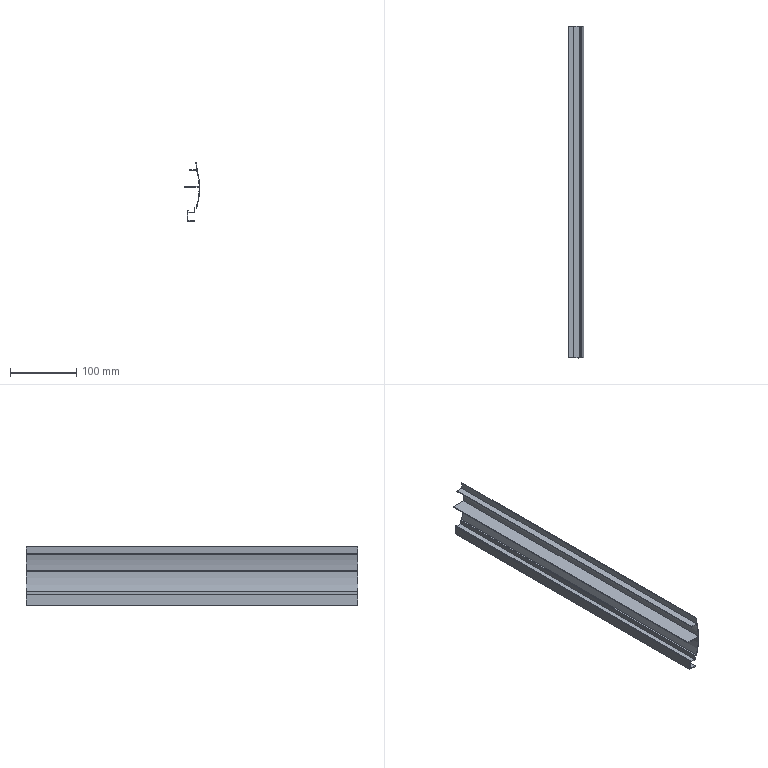Component | SolidWorks | Blade-17 | 1 solid | 27 faces | box 23.47 x 500 x 87.98 mm | volume 81818 mm3 | plane 24 | cylinder 3 | commonest cylinder face diameters 190.922 x3
build123d program:
from build123d import *

# Parameters (mm, degrees)
BOSS_EXTRUDE1_DEPTH = 500


with BuildPart() as part:
    # Sketch1 → Boss-Extrude1 (new body)
    with BuildSketch(Plane.XY):
        with BuildLine():
            Line((52.448, 10.612), (52.448, -5.008))
            Line((52.448, -5.008), (51.164, -5.008))
            Line((51.164, -5.008), (51.164, 10.227))
            Line((51.164, 10.227), (51.164, 17.359))
            ThreePointArc((51.164, 17.359), (35.594, 16.542), (20.364, 13.201))
            Line((20.364, 13.201), (20.364, 10.4))
            Line((20.364, 10.4), (13.6, 10.4))
            Line((13.6, 10.4), (13.6, 1.1))
            Line((13.6, 1.1), (15.3, 1.1))
            Line((15.3, 1.1), (15.3, 0))
            Line((15.3, 0), (0, 0))
            Line((0, 0), (0, 11.2))
            Line((0, 11.2), (1.1, 11.2))
            Line((1.1, 11.2), (1.1, 1.1))
            Line((1.1, 1.1), (12.5, 1.1))
            Line((12.5, 1.1), (12.5, 11.5))
            Line((12.5, 11.5), (19.4, 11.5))
            Line((19.4, 11.5), (19.4, 14))
            ThreePointArc((19.4, 14), (48.454, 18.5), (77.5, 13.945))
            Line((77.5, 13.945), (88, 12.9))
            Line((88, 12.9), (88, 11.8))
            Line((88, 11.8), (77.5, 12.9))
            Line((77.5, 12.9), (77.5, 2.6))
            Line((77.5, 2.6), (76.4, 2.6))
            Line((76.4, 2.6), (76.4, 13.19))
            ThreePointArc((76.4, 13.19), (64.556, 16.017), (52.448, 17.313))
            Line((52.448, 17.313), (52.448, 10.612))
        make_face()
    extrude(amount=BOSS_EXTRUDE1_DEPTH)


solid = part.part

# Placed as in the assembly
solid = solid.moved(Location((101.142, 41.806, 695.913), (-90, 0, -89.089)))
STEP:
#1=COLOUR_RGB('',0.7922,0.8196,0.9333);
#2=FILL_AREA_STYLE_COLOUR('',#1);
#3=FILL_AREA_STYLE('',(#2));
#4=SURFACE_STYLE_FILL_AREA(#3);
#5=SURFACE_SIDE_STYLE('',(#4));
#6=SURFACE_STYLE_USAGE(.BOTH.,#5);
#7=PRESENTATION_STYLE_ASSIGNMENT((#6));
#8=CARTESIAN_POINT('',(4.549,1.646,30.397));
#9=VERTEX_POINT('',#8);
#10=CARTESIAN_POINT('',(4.696,1.646,29.452));
#11=VERTEX_POINT('',#10);
#12=CARTESIAN_POINT('',(0.9394,1.646,29.351));
#13=DIRECTION('',(-0.,1.,0.));
#14=DIRECTION('',(0.0159,-0.,0.9999));
#15=AXIS2_PLACEMENT_3D('',#12,#13,#14);
#16=CIRCLE('',#15,3.758);
#17=EDGE_CURVE('',#9,#11,#16,.T.);
#18=ORIENTED_EDGE('',*,*,#17,.F.);
#19=CARTESIAN_POINT('',(4.549,21.331,30.397));
#20=VERTEX_POINT('',#19);
#21=CARTESIAN_POINT('',(4.549,21.331,30.397));
#22=DIRECTION('',(0.,-1.,-0.));
#23=VECTOR('',#22,39.37);
#24=LINE('',#21,#23);
#25=EDGE_CURVE('',#20,#9,#24,.T.);
#26=ORIENTED_EDGE('',*,*,#25,.F.);
#27=CARTESIAN_POINT('',(4.696,21.331,29.452));
#28=VERTEX_POINT('',#27);
#29=CARTESIAN_POINT('',(0.9394,21.331,29.351));
#30=DIRECTION('',(-0.,1.,0.));
#31=DIRECTION('',(0.0159,0.,0.9999));
#32=AXIS2_PLACEMENT_3D('',#29,#30,#31);
#33=CIRCLE('',#32,3.758);
#34=EDGE_CURVE('',#20,#28,#33,.T.);
#35=ORIENTED_EDGE('',*,*,#34,.T.);
#36=CARTESIAN_POINT('',(4.696,21.331,29.452));
#37=DIRECTION('',(0.,-1.,-0.));
#38=VECTOR('',#37,39.37);
#39=LINE('',#36,#38);
#40=EDGE_CURVE('',#28,#11,#39,.T.);
#41=ORIENTED_EDGE('',*,*,#40,.T.);
#42=EDGE_LOOP('',(#18,#26,#35,#41));
#43=FACE_OUTER_BOUND('',#42,.T.);
#44=CARTESIAN_POINT('',(0.9394,21.331,29.351));
#45=DIRECTION('',(0.,-1.,-0.));
#46=DIRECTION('',(-0.0159,0.,-0.9999));
#47=AXIS2_PLACEMENT_3D('',#44,#45,#46);
#48=CYLINDRICAL_SURFACE('',#47,3.758);
#49=ADVANCED_FACE('',(#43),#48,.F.);
#50=CARTESIAN_POINT('',(4.132,1.646,30.404));
#51=VERTEX_POINT('',#50);
#52=CARTESIAN_POINT('',(4.549,1.646,30.397));
#53=DIRECTION('',(-0.9999,-0.,0.0159));
#54=VECTOR('',#53,39.37);
#55=LINE('',#52,#54);
#56=EDGE_CURVE('',#9,#51,#55,.T.);
#57=ORIENTED_EDGE('',*,*,#56,.T.);
#58=CARTESIAN_POINT('',(4.132,21.331,30.404));
#59=VERTEX_POINT('',#58);
#60=CARTESIAN_POINT('',(4.132,21.331,30.404));
#61=DIRECTION('',(0.,-1.,-0.));
#62=VECTOR('',#61,39.37);
#63=LINE('',#60,#62);
#64=EDGE_CURVE('',#59,#51,#63,.T.);
#65=ORIENTED_EDGE('',*,*,#64,.F.);
#66=CARTESIAN_POINT('',(4.549,21.331,30.397));
#67=DIRECTION('',(-0.9999,-0.,0.0159));
#68=VECTOR('',#67,39.37);
#69=LINE('',#66,#68);
#70=EDGE_CURVE('',#20,#59,#69,.T.);
#71=ORIENTED_EDGE('',*,*,#70,.F.);
#72=ORIENTED_EDGE('',*,*,#25,.T.);
#73=EDGE_LOOP('',(#57,#65,#71,#72));
#74=FACE_OUTER_BOUND('',#73,.T.);
#75=CARTESIAN_POINT('',(4.549,21.331,30.397));
#76=DIRECTION('',(0.0159,-0.,0.9999));
#77=DIRECTION('',(0.,-1.,-0.));
#78=AXIS2_PLACEMENT_3D('',#75,#76,#77);
#79=PLANE('',#78);
#80=ADVANCED_FACE('',(#74),#79,.F.);
#81=CARTESIAN_POINT('',(4.133,1.646,30.447));
#82=VERTEX_POINT('',#81);
#83=CARTESIAN_POINT('',(4.132,1.646,30.404));
#84=DIRECTION('',(0.0159,-0.,0.9999));
#85=VECTOR('',#84,39.37);
#86=LINE('',#83,#85);
#87=EDGE_CURVE('',#51,#82,#86,.T.);
#88=ORIENTED_EDGE('',*,*,#87,.T.);
#89=CARTESIAN_POINT('',(4.133,21.331,30.447));
#90=VERTEX_POINT('',#89);
#91=CARTESIAN_POINT('',(4.133,21.331,30.447));
#92=DIRECTION('',(0.,-1.,-0.));
#93=VECTOR('',#92,39.37);
#94=LINE('',#91,#93);
#95=EDGE_CURVE('',#90,#82,#94,.T.);
#96=ORIENTED_EDGE('',*,*,#95,.F.);
#97=CARTESIAN_POINT('',(4.132,21.331,30.404));
#98=DIRECTION('',(0.0159,-0.,0.9999));
#99=VECTOR('',#98,39.37);
#100=LINE('',#97,#99);
#101=EDGE_CURVE('',#59,#90,#100,.T.);
#102=ORIENTED_EDGE('',*,*,#101,.F.);
#103=ORIENTED_EDGE('',*,*,#64,.T.);
#104=EDGE_LOOP('',(#88,#96,#102,#103));
#105=FACE_OUTER_BOUND('',#104,.T.);
#106=CARTESIAN_POINT('',(4.132,21.331,30.404));
#107=DIRECTION('',(0.9999,0.,-0.0159));
#108=DIRECTION('',(-0.,1.,0.));
#109=AXIS2_PLACEMENT_3D('',#106,#107,#108);
#110=PLANE('',#109);
#111=ADVANCED_FACE('',(#105),#110,.F.);
#112=CARTESIAN_POINT('',(4.538,1.646,30.441));
#113=VERTEX_POINT('',#112);
#114=CARTESIAN_POINT('',(4.133,1.646,30.447));
#115=DIRECTION('',(0.9999,0.,-0.0159));
#116=VECTOR('',#115,39.37);
#117=LINE('',#114,#116);
#118=EDGE_CURVE('',#82,#113,#117,.T.);
#119=ORIENTED_EDGE('',*,*,#118,.T.);
#120=CARTESIAN_POINT('',(4.538,21.331,30.441));
#121=VERTEX_POINT('',#120);
#122=CARTESIAN_POINT('',(4.538,21.331,30.441));
#123=DIRECTION('',(0.,-1.,-0.));
#124=VECTOR('',#123,39.37);
#125=LINE('',#122,#124);
#126=EDGE_CURVE('',#121,#113,#125,.T.);
#127=ORIENTED_EDGE('',*,*,#126,.F.);
#128=CARTESIAN_POINT('',(4.133,21.331,30.447));
#129=DIRECTION('',(0.9999,0.,-0.0159));
#130=VECTOR('',#129,39.37);
#131=LINE('',#128,#130);
#132=EDGE_CURVE('',#90,#121,#131,.T.);
#133=ORIENTED_EDGE('',*,*,#132,.F.);
#134=ORIENTED_EDGE('',*,*,#95,.T.);
#135=EDGE_LOOP('',(#119,#127,#133,#134));
#136=FACE_OUTER_BOUND('',#135,.T.);
#137=CARTESIAN_POINT('',(4.133,21.331,30.447));
#138=DIRECTION('',(-0.0159,0.,-0.9999));
#139=DIRECTION('',(-0.,1.,0.));
#140=AXIS2_PLACEMENT_3D('',#137,#138,#139);
#141=PLANE('',#140);
#142=ADVANCED_FACE('',(#136),#141,.F.);
#143=CARTESIAN_POINT('',(4.502,1.646,30.855));
#144=VERTEX_POINT('',#143);
#145=CARTESIAN_POINT('',(4.538,1.646,30.441));
#146=DIRECTION('',(-0.08837,-0.,0.9961));
#147=VECTOR('',#146,39.37);
#148=LINE('',#145,#147);
#149=EDGE_CURVE('',#113,#144,#148,.T.);
#150=ORIENTED_EDGE('',*,*,#149,.T.);
#151=CARTESIAN_POINT('',(4.502,21.331,30.855));
#152=VERTEX_POINT('',#151);
#153=CARTESIAN_POINT('',(4.502,21.331,30.855));
#154=DIRECTION('',(0.,-1.,-0.));
#155=VECTOR('',#154,39.37);
#156=LINE('',#153,#155);
#157=EDGE_CURVE('',#152,#144,#156,.T.);
#158=ORIENTED_EDGE('',*,*,#157,.F.);
#159=CARTESIAN_POINT('',(4.538,21.331,30.441));
#160=DIRECTION('',(-0.08837,-0.,0.9961));
#161=VECTOR('',#160,39.37);
#162=LINE('',#159,#161);
#163=EDGE_CURVE('',#121,#152,#162,.T.);
#164=ORIENTED_EDGE('',*,*,#163,.F.);
#165=ORIENTED_EDGE('',*,*,#126,.T.);
#166=EDGE_LOOP('',(#150,#158,#164,#165));
#167=FACE_OUTER_BOUND('',#166,.T.);
#168=CARTESIAN_POINT('',(4.538,21.331,30.441));
#169=DIRECTION('',(0.9961,0.,0.08837));
#170=DIRECTION('',(0.08837,0.,-0.9961));
#171=AXIS2_PLACEMENT_3D('',#168,#169,#170);
#172=PLANE('',#171);
#173=ADVANCED_FACE('',(#167),#172,.F.);
#174=CARTESIAN_POINT('',(4.545,1.646,30.854));
#175=VERTEX_POINT('',#174);
#176=CARTESIAN_POINT('',(4.502,1.646,30.855));
#177=DIRECTION('',(0.9999,0.,-0.0159));
#178=VECTOR('',#177,39.37);
#179=LINE('',#176,#178);
#180=EDGE_CURVE('',#144,#175,#179,.T.);
#181=ORIENTED_EDGE('',*,*,#180,.T.);
#182=CARTESIAN_POINT('',(4.545,21.331,30.854));
#183=VERTEX_POINT('',#182);
#184=CARTESIAN_POINT('',(4.545,21.331,30.854));
#185=DIRECTION('',(0.,-1.,-0.));
#186=VECTOR('',#185,39.37);
#187=LINE('',#184,#186);
#188=EDGE_CURVE('',#183,#175,#187,.T.);
#189=ORIENTED_EDGE('',*,*,#188,.F.);
#190=CARTESIAN_POINT('',(4.502,21.331,30.855));
#191=DIRECTION('',(0.9999,0.,-0.0159));
#192=VECTOR('',#191,39.37);
#193=LINE('',#190,#192);
#194=EDGE_CURVE('',#152,#183,#193,.T.);
#195=ORIENTED_EDGE('',*,*,#194,.F.);
#196=ORIENTED_EDGE('',*,*,#157,.T.);
#197=EDGE_LOOP('',(#181,#189,#195,#196));
#198=FACE_OUTER_BOUND('',#197,.T.);
#199=CARTESIAN_POINT('',(4.502,21.331,30.855));
#200=DIRECTION('',(-0.0159,0.,-0.9999));
#201=DIRECTION('',(-0.,1.,0.));
#202=AXIS2_PLACEMENT_3D('',#199,#200,#201);
#203=PLANE('',#202);
#204=ADVANCED_FACE('',(#198),#203,.F.);
#205=CARTESIAN_POINT('',(4.579,1.646,30.44));
#206=VERTEX_POINT('',#205);
#207=CARTESIAN_POINT('',(4.545,1.646,30.854));
#208=DIRECTION('',(0.08323,0.,-0.9965));
#209=VECTOR('',#208,39.37);
#210=LINE('',#207,#209);
#211=EDGE_CURVE('',#175,#206,#210,.T.);
#212=ORIENTED_EDGE('',*,*,#211,.T.);
#213=CARTESIAN_POINT('',(4.579,21.331,30.44));
#214=VERTEX_POINT('',#213);
#215=CARTESIAN_POINT('',(4.579,21.331,30.44));
#216=DIRECTION('',(0.,-1.,-0.));
#217=VECTOR('',#216,39.37);
#218=LINE('',#215,#217);
#219=EDGE_CURVE('',#214,#206,#218,.T.);
#220=ORIENTED_EDGE('',*,*,#219,.F.);
#221=CARTESIAN_POINT('',(4.545,21.331,30.854));
#222=DIRECTION('',(0.08323,0.,-0.9965));
#223=VECTOR('',#222,39.37);
#224=LINE('',#221,#223);
#225=EDGE_CURVE('',#183,#214,#224,.T.);
#226=ORIENTED_EDGE('',*,*,#225,.F.);
#227=ORIENTED_EDGE('',*,*,#188,.T.);
#228=EDGE_LOOP('',(#212,#220,#226,#227));
#229=FACE_OUTER_BOUND('',#228,.T.);
#230=CARTESIAN_POINT('',(4.545,21.331,30.854));
#231=DIRECTION('',(-0.9965,-0.,-0.08323));
#232=DIRECTION('',(-0.08323,-0.,0.9965));
#233=AXIS2_PLACEMENT_3D('',#230,#231,#232);
#234=PLANE('',#233);
#235=ADVANCED_FACE('',(#229),#234,.F.);
#236=CARTESIAN_POINT('',(4.545,1.646,28.153));
#237=VERTEX_POINT('',#236);
#238=CARTESIAN_POINT('',(0.9827,1.646,29.35));
#239=DIRECTION('',(-0.,1.,0.));
#240=DIRECTION('',(0.0159,-0.,0.9999));
#241=AXIS2_PLACEMENT_3D('',#238,#239,#240);
#242=CIRCLE('',#241,3.758);
#243=EDGE_CURVE('',#206,#237,#242,.T.);
#244=ORIENTED_EDGE('',*,*,#243,.T.);
#245=CARTESIAN_POINT('',(4.545,21.331,28.153));
#246=VERTEX_POINT('',#245);
#247=CARTESIAN_POINT('',(4.545,21.331,28.153));
#248=DIRECTION('',(0.,-1.,-0.));
#249=VECTOR('',#248,39.37);
#250=LINE('',#247,#249);
#251=EDGE_CURVE('',#246,#237,#250,.T.);
#252=ORIENTED_EDGE('',*,*,#251,.F.);
#253=CARTESIAN_POINT('',(0.9827,21.331,29.35));
#254=DIRECTION('',(-0.,1.,0.));
#255=DIRECTION('',(0.0159,0.,0.9999));
#256=AXIS2_PLACEMENT_3D('',#253,#254,#255);
#257=CIRCLE('',#256,3.758);
#258=EDGE_CURVE('',#214,#246,#257,.T.);
#259=ORIENTED_EDGE('',*,*,#258,.F.);
#260=ORIENTED_EDGE('',*,*,#219,.T.);
#261=EDGE_LOOP('',(#244,#252,#259,#260));
#262=FACE_OUTER_BOUND('',#261,.T.);
#263=CARTESIAN_POINT('',(0.9827,21.331,29.35));
#264=DIRECTION('',(0.,-1.,-0.));
#265=DIRECTION('',(-0.0159,0.,-0.9999));
#266=AXIS2_PLACEMENT_3D('',#263,#264,#265);
#267=CYLINDRICAL_SURFACE('',#266,3.758);
#268=ADVANCED_FACE('',(#262),#267,.T.);
#269=CARTESIAN_POINT('',(4.447,1.646,28.155));
#270=VERTEX_POINT('',#269);
#271=CARTESIAN_POINT('',(4.545,1.646,28.153));
#272=DIRECTION('',(-0.9999,-0.,0.0159));
#273=VECTOR('',#272,39.37);
#274=LINE('',#271,#273);
#275=EDGE_CURVE('',#237,#270,#274,.T.);
#276=ORIENTED_EDGE('',*,*,#275,.T.);
#277=CARTESIAN_POINT('',(4.447,21.331,28.155));
#278=VERTEX_POINT('',#277);
#279=CARTESIAN_POINT('',(4.447,21.331,28.155));
#280=DIRECTION('',(0.,-1.,-0.));
#281=VECTOR('',#280,39.37);
#282=LINE('',#279,#281);
#283=EDGE_CURVE('',#278,#270,#282,.T.);
#284=ORIENTED_EDGE('',*,*,#283,.F.);
#285=CARTESIAN_POINT('',(4.545,21.331,28.153));
#286=DIRECTION('',(-0.9999,-0.,0.0159));
#287=VECTOR('',#286,39.37);
#288=LINE('',#285,#287);
#289=EDGE_CURVE('',#246,#278,#288,.T.);
#290=ORIENTED_EDGE('',*,*,#289,.F.);
#291=ORIENTED_EDGE('',*,*,#251,.T.);
#292=EDGE_LOOP('',(#276,#284,#290,#291));
#293=FACE_OUTER_BOUND('',#292,.T.);
#294=CARTESIAN_POINT('',(4.545,21.331,28.153));
#295=DIRECTION('',(0.0159,-0.,0.9999));
#296=DIRECTION('',(0.,-1.,-0.));
#297=AXIS2_PLACEMENT_3D('',#294,#295,#296);
#298=PLANE('',#297);
#299=ADVANCED_FACE('',(#293),#298,.F.);
#300=CARTESIAN_POINT('',(4.442,1.646,27.883));
#301=VERTEX_POINT('',#300);
#302=CARTESIAN_POINT('',(4.447,1.646,28.155));
#303=DIRECTION('',(-0.0159,0.,-0.9999));
#304=VECTOR('',#303,39.37);
#305=LINE('',#302,#304);
#306=EDGE_CURVE('',#270,#301,#305,.T.);
#307=ORIENTED_EDGE('',*,*,#306,.T.);
#308=CARTESIAN_POINT('',(4.442,21.331,27.883));
#309=VERTEX_POINT('',#308);
#310=CARTESIAN_POINT('',(4.442,21.331,27.883));
#311=DIRECTION('',(0.,-1.,-0.));
#312=VECTOR('',#311,39.37);
#313=LINE('',#310,#312);
#314=EDGE_CURVE('',#309,#301,#313,.T.);
#315=ORIENTED_EDGE('',*,*,#314,.F.);
#316=CARTESIAN_POINT('',(4.447,21.331,28.155));
#317=DIRECTION('',(-0.0159,0.,-0.9999));
#318=VECTOR('',#317,39.37);
#319=LINE('',#316,#318);
#320=EDGE_CURVE('',#278,#309,#319,.T.);
#321=ORIENTED_EDGE('',*,*,#320,.F.);
#322=ORIENTED_EDGE('',*,*,#283,.T.);
#323=EDGE_LOOP('',(#307,#315,#321,#322));
#324=FACE_OUTER_BOUND('',#323,.T.);
#325=CARTESIAN_POINT('',(4.447,21.331,28.155));
#326=DIRECTION('',(-0.9999,-0.,0.0159));
#327=DIRECTION('',(0.,-1.,-0.));
#328=AXIS2_PLACEMENT_3D('',#325,#326,#327);
#329=PLANE('',#328);
#330=ADVANCED_FACE('',(#324),#329,.F.);
#331=CARTESIAN_POINT('',(4.033,1.646,27.89));
#332=VERTEX_POINT('',#331);
#333=CARTESIAN_POINT('',(4.442,1.646,27.883));
#334=DIRECTION('',(-0.9999,-0.,0.0159));
#335=VECTOR('',#334,39.37);
#336=LINE('',#333,#335);
#337=EDGE_CURVE('',#301,#332,#336,.T.);
#338=ORIENTED_EDGE('',*,*,#337,.T.);
#339=CARTESIAN_POINT('',(4.033,21.331,27.89));
#340=VERTEX_POINT('',#339);
#341=CARTESIAN_POINT('',(4.033,21.331,27.89));
#342=DIRECTION('',(0.,-1.,-0.));
#343=VECTOR('',#342,39.37);
#344=LINE('',#341,#343);
#345=EDGE_CURVE('',#340,#332,#344,.T.);
#346=ORIENTED_EDGE('',*,*,#345,.F.);
#347=CARTESIAN_POINT('',(4.442,21.331,27.883));
#348=DIRECTION('',(-0.9999,-0.,0.0159));
#349=VECTOR('',#348,39.37);
#350=LINE('',#347,#349);
#351=EDGE_CURVE('',#309,#340,#350,.T.);
#352=ORIENTED_EDGE('',*,*,#351,.F.);
#353=ORIENTED_EDGE('',*,*,#314,.T.);
#354=EDGE_LOOP('',(#338,#346,#352,#353));
#355=FACE_OUTER_BOUND('',#354,.T.);
#356=CARTESIAN_POINT('',(4.442,21.331,27.883));
#357=DIRECTION('',(0.0159,-0.,0.9999));
#358=DIRECTION('',(0.,-1.,-0.));
#359=AXIS2_PLACEMENT_3D('',#356,#357,#358);
#360=PLANE('',#359);
#361=ADVANCED_FACE('',(#355),#360,.F.);
#362=CARTESIAN_POINT('',(4.026,1.646,27.441));
#363=VERTEX_POINT('',#362);
#364=CARTESIAN_POINT('',(4.033,1.646,27.89));
#365=DIRECTION('',(-0.0159,0.,-0.9999));
#366=VECTOR('',#365,39.37);
#367=LINE('',#364,#366);
#368=EDGE_CURVE('',#332,#363,#367,.T.);
#369=ORIENTED_EDGE('',*,*,#368,.T.);
#370=CARTESIAN_POINT('',(4.026,21.331,27.441));
#371=VERTEX_POINT('',#370);
#372=CARTESIAN_POINT('',(4.026,21.331,27.441));
#373=DIRECTION('',(0.,-1.,-0.));
#374=VECTOR('',#373,39.37);
#375=LINE('',#372,#374);
#376=EDGE_CURVE('',#371,#363,#375,.T.);
#377=ORIENTED_EDGE('',*,*,#376,.F.);
#378=CARTESIAN_POINT('',(4.033,21.331,27.89));
#379=DIRECTION('',(-0.0159,0.,-0.9999));
#380=VECTOR('',#379,39.37);
#381=LINE('',#378,#380);
#382=EDGE_CURVE('',#340,#371,#381,.T.);
#383=ORIENTED_EDGE('',*,*,#382,.F.);
#384=ORIENTED_EDGE('',*,*,#345,.T.);
#385=EDGE_LOOP('',(#369,#377,#383,#384));
#386=FACE_OUTER_BOUND('',#385,.T.);
#387=CARTESIAN_POINT('',(4.033,21.331,27.89));
#388=DIRECTION('',(-0.9999,-0.,0.0159));
#389=DIRECTION('',(0.,-1.,-0.));
#390=AXIS2_PLACEMENT_3D('',#387,#388,#389);
#391=PLANE('',#390);
#392=ADVANCED_FACE('',(#386),#391,.F.);
#393=CARTESIAN_POINT('',(4.424,1.646,27.434));
#394=VERTEX_POINT('',#393);
#395=CARTESIAN_POINT('',(4.026,1.646,27.441));
#396=DIRECTION('',(0.9999,0.,-0.0159));
#397=VECTOR('',#396,39.37);
#398=LINE('',#395,#397);
#399=EDGE_CURVE('',#363,#394,#398,.T.);
#400=ORIENTED_EDGE('',*,*,#399,.T.);
#401=CARTESIAN_POINT('',(4.424,21.331,27.434));
#402=VERTEX_POINT('',#401);
#403=CARTESIAN_POINT('',(4.424,21.331,27.434));
#404=DIRECTION('',(0.,-1.,-0.));
#405=VECTOR('',#404,39.37);
#406=LINE('',#403,#405);
#407=EDGE_CURVE('',#402,#394,#406,.T.);
#408=ORIENTED_EDGE('',*,*,#407,.F.);
#409=CARTESIAN_POINT('',(4.026,21.331,27.441));
#410=DIRECTION('',(0.9999,0.,-0.0159));
#411=VECTOR('',#410,39.37);
#412=LINE('',#409,#411);
#413=EDGE_CURVE('',#371,#402,#412,.T.);
#414=ORIENTED_EDGE('',*,*,#413,.F.);
#415=ORIENTED_EDGE('',*,*,#376,.T.);
#416=EDGE_LOOP('',(#400,#408,#414,#415));
#417=FACE_OUTER_BOUND('',#416,.T.);
#418=CARTESIAN_POINT('',(4.026,21.331,27.441));
#419=DIRECTION('',(-0.0159,0.,-0.9999));
#420=DIRECTION('',(-0.,1.,0.));
#421=AXIS2_PLACEMENT_3D('',#418,#419,#420);
#422=PLANE('',#421);
#423=ADVANCED_FACE('',(#417),#422,.F.);
#424=CARTESIAN_POINT('',(4.423,1.646,27.391));
#425=VERTEX_POINT('',#424);
#426=CARTESIAN_POINT('',(4.424,1.646,27.434));
#427=DIRECTION('',(-0.0159,0.,-0.9999));
#428=VECTOR('',#427,39.37);
#429=LINE('',#426,#428);
#430=EDGE_CURVE('',#394,#425,#429,.T.);
#431=ORIENTED_EDGE('',*,*,#430,.T.);
#432=CARTESIAN_POINT('',(4.423,21.331,27.391));
#433=VERTEX_POINT('',#432);
#434=CARTESIAN_POINT('',(4.423,21.331,27.391));
#435=DIRECTION('',(0.,-1.,-0.));
#436=VECTOR('',#435,39.37);
#437=LINE('',#434,#436);
#438=EDGE_CURVE('',#433,#425,#437,.T.);
#439=ORIENTED_EDGE('',*,*,#438,.F.);
#440=CARTESIAN_POINT('',(4.424,21.331,27.434));
#441=DIRECTION('',(-0.0159,0.,-0.9999));
#442=VECTOR('',#441,39.37);
#443=LINE('',#440,#442);
#444=EDGE_CURVE('',#402,#433,#443,.T.);
#445=ORIENTED_EDGE('',*,*,#444,.F.);
#446=ORIENTED_EDGE('',*,*,#407,.T.);
#447=EDGE_LOOP('',(#431,#439,#445,#446));
#448=FACE_OUTER_BOUND('',#447,.T.);
#449=CARTESIAN_POINT('',(4.424,21.331,27.434));
#450=DIRECTION('',(-0.9999,-0.,0.0159));
#451=DIRECTION('',(0.,-1.,-0.));
#452=AXIS2_PLACEMENT_3D('',#449,#450,#451);
#453=PLANE('',#452);
#454=ADVANCED_FACE('',(#448),#453,.F.);
#455=CARTESIAN_POINT('',(3.982,1.646,27.398));
#456=VERTEX_POINT('',#455);
#457=CARTESIAN_POINT('',(4.423,1.646,27.391));
#458=DIRECTION('',(-0.9999,-0.,0.0159));
#459=VECTOR('',#458,39.37);
#460=LINE('',#457,#459);
#461=EDGE_CURVE('',#425,#456,#460,.T.);
#462=ORIENTED_EDGE('',*,*,#461,.T.);
#463=CARTESIAN_POINT('',(3.982,21.331,27.398));
#464=VERTEX_POINT('',#463);
#465=CARTESIAN_POINT('',(3.982,21.331,27.398));
#466=DIRECTION('',(0.,-1.,-0.));
#467=VECTOR('',#466,39.37);
#468=LINE('',#465,#467);
#469=EDGE_CURVE('',#464,#456,#468,.T.);
#470=ORIENTED_EDGE('',*,*,#469,.F.);
#471=CARTESIAN_POINT('',(4.423,21.331,27.391));
#472=DIRECTION('',(-0.9999,-0.,0.0159));
#473=VECTOR('',#472,39.37);
#474=LINE('',#471,#473);
#475=EDGE_CURVE('',#433,#464,#474,.T.);
#476=ORIENTED_EDGE('',*,*,#475,.F.);
#477=ORIENTED_EDGE('',*,*,#438,.T.);
#478=EDGE_LOOP('',(#462,#470,#476,#477));
#479=FACE_OUTER_BOUND('',#478,.T.);
#480=CARTESIAN_POINT('',(4.423,21.331,27.391));
#481=DIRECTION('',(0.0159,-0.,0.9999));
#482=DIRECTION('',(0.,-1.,-0.));
#483=AXIS2_PLACEMENT_3D('',#480,#481,#482);
#484=PLANE('',#483);
#485=ADVANCED_FACE('',(#479),#484,.F.);
#486=CARTESIAN_POINT('',(3.992,1.646,28.));
#487=VERTEX_POINT('',#486);
#488=CARTESIAN_POINT('',(3.982,1.646,27.398));
#489=DIRECTION('',(0.0159,-0.,0.9999));
#490=VECTOR('',#489,39.37);
#491=LINE('',#488,#490);
#492=EDGE_CURVE('',#456,#487,#491,.T.);
#493=ORIENTED_EDGE('',*,*,#492,.T.);
#494=CARTESIAN_POINT('',(3.992,21.331,28.));
#495=VERTEX_POINT('',#494);
#496=CARTESIAN_POINT('',(3.992,21.331,28.));
#497=DIRECTION('',(0.,-1.,-0.));
#498=VECTOR('',#497,39.37);
#499=LINE('',#496,#498);
#500=EDGE_CURVE('',#495,#487,#499,.T.);
#501=ORIENTED_EDGE('',*,*,#500,.F.);
#502=CARTESIAN_POINT('',(3.982,21.331,27.398));
#503=DIRECTION('',(0.0159,-0.,0.9999));
#504=VECTOR('',#503,39.37);
#505=LINE('',#502,#504);
#506=EDGE_CURVE('',#464,#495,#505,.T.);
#507=ORIENTED_EDGE('',*,*,#506,.F.);
#508=ORIENTED_EDGE('',*,*,#469,.T.);
#509=EDGE_LOOP('',(#493,#501,#507,#508));
#510=FACE_OUTER_BOUND('',#509,.T.);
#511=CARTESIAN_POINT('',(3.982,21.331,27.398));
#512=DIRECTION('',(0.9999,0.,-0.0159));
#513=DIRECTION('',(-0.,1.,0.));
#514=AXIS2_PLACEMENT_3D('',#511,#512,#513);
#515=PLANE('',#514);
#516=ADVANCED_FACE('',(#510),#515,.F.);
#517=CARTESIAN_POINT('',(4.035,1.646,28.));
#518=VERTEX_POINT('',#517);
#519=CARTESIAN_POINT('',(3.992,1.646,28.));
#520=DIRECTION('',(0.9999,0.,-0.0159));
#521=VECTOR('',#520,39.37);
#522=LINE('',#519,#521);
#523=EDGE_CURVE('',#487,#518,#522,.T.);
#524=ORIENTED_EDGE('',*,*,#523,.T.);
#525=CARTESIAN_POINT('',(4.035,21.331,28.));
#526=VERTEX_POINT('',#525);
#527=CARTESIAN_POINT('',(4.035,21.331,28.));
#528=DIRECTION('',(0.,-1.,-0.));
#529=VECTOR('',#528,39.37);
#530=LINE('',#527,#529);
#531=EDGE_CURVE('',#526,#518,#530,.T.);
#532=ORIENTED_EDGE('',*,*,#531,.F.);
#533=CARTESIAN_POINT('',(3.992,21.331,28.));
#534=DIRECTION('',(0.9999,0.,-0.0159));
#535=VECTOR('',#534,39.37);
#536=LINE('',#533,#535);
#537=EDGE_CURVE('',#495,#526,#536,.T.);
#538=ORIENTED_EDGE('',*,*,#537,.F.);
#539=ORIENTED_EDGE('',*,*,#500,.T.);
#540=EDGE_LOOP('',(#524,#532,#538,#539));
#541=FACE_OUTER_BOUND('',#540,.T.);
#542=CARTESIAN_POINT('',(3.992,21.331,28.));
#543=DIRECTION('',(-0.0159,0.,-0.9999));
#544=DIRECTION('',(-0.,1.,0.));
#545=AXIS2_PLACEMENT_3D('',#542,#543,#544);
#546=PLANE('',#545);
#547=ADVANCED_FACE('',(#541),#546,.F.);
#548=CARTESIAN_POINT('',(4.034,1.646,27.933));
#549=VERTEX_POINT('',#548);
#550=CARTESIAN_POINT('',(4.035,1.646,28.));
#551=DIRECTION('',(-0.0159,0.,-0.9999));
#552=VECTOR('',#551,39.37);
#553=LINE('',#550,#552);
#554=EDGE_CURVE('',#518,#549,#553,.T.);
#555=ORIENTED_EDGE('',*,*,#554,.T.);
#556=CARTESIAN_POINT('',(4.034,21.331,27.933));
#557=VERTEX_POINT('',#556);
#558=CARTESIAN_POINT('',(4.034,21.331,27.933));
#559=DIRECTION('',(0.,-1.,-0.));
#560=VECTOR('',#559,39.37);
#561=LINE('',#558,#560);
#562=EDGE_CURVE('',#557,#549,#561,.T.);
#563=ORIENTED_EDGE('',*,*,#562,.F.);
#564=CARTESIAN_POINT('',(4.035,21.331,28.));
#565=DIRECTION('',(-0.0159,0.,-0.9999));
#566=VECTOR('',#565,39.37);
#567=LINE('',#564,#566);
#568=EDGE_CURVE('',#526,#557,#567,.T.);
#569=ORIENTED_EDGE('',*,*,#568,.F.);
#570=ORIENTED_EDGE('',*,*,#531,.T.);
#571=EDGE_LOOP('',(#555,#563,#569,#570));
#572=FACE_OUTER_BOUND('',#571,.T.);
#573=CARTESIAN_POINT('',(4.035,21.331,28.));
#574=DIRECTION('',(-0.9999,-0.,0.0159));
#575=DIRECTION('',(0.,-1.,-0.));
#576=AXIS2_PLACEMENT_3D('',#573,#574,#575);
#577=PLANE('',#576);
#578=ADVANCED_FACE('',(#572),#577,.F.);
#579=CARTESIAN_POINT('',(4.4,1.646,27.927));
#580=VERTEX_POINT('',#579);
#581=CARTESIAN_POINT('',(4.034,1.646,27.933));
#582=DIRECTION('',(0.9999,0.,-0.0159));
#583=VECTOR('',#582,39.37);
#584=LINE('',#581,#583);
#585=EDGE_CURVE('',#549,#580,#584,.T.);
#586=ORIENTED_EDGE('',*,*,#585,.T.);
#587=CARTESIAN_POINT('',(4.4,21.331,27.927));
#588=VERTEX_POINT('',#587);
#589=CARTESIAN_POINT('',(4.4,21.331,27.927));
#590=DIRECTION('',(0.,-1.,-0.));
#591=VECTOR('',#590,39.37);
#592=LINE('',#589,#591);
#593=EDGE_CURVE('',#588,#580,#592,.T.);
#594=ORIENTED_EDGE('',*,*,#593,.F.);
#595=CARTESIAN_POINT('',(4.034,21.331,27.933));
#596=DIRECTION('',(0.9999,0.,-0.0159));
#597=VECTOR('',#596,39.37);
#598=LINE('',#595,#597);
#599=EDGE_CURVE('',#557,#588,#598,.T.);
#600=ORIENTED_EDGE('',*,*,#599,.F.);
#601=ORIENTED_EDGE('',*,*,#562,.T.);
#602=EDGE_LOOP('',(#586,#594,#600,#601));
#603=FACE_OUTER_BOUND('',#602,.T.);
#604=CARTESIAN_POINT('',(4.034,21.331,27.933));
#605=DIRECTION('',(-0.0159,0.,-0.9999));
#606=DIRECTION('',(-0.,1.,0.));
#607=AXIS2_PLACEMENT_3D('',#604,#605,#606);
#608=PLANE('',#607);
#609=ADVANCED_FACE('',(#603),#608,.F.);
#610=CARTESIAN_POINT('',(4.404,1.646,28.193));
#611=VERTEX_POINT('',#610);
#612=CARTESIAN_POINT('',(4.4,1.646,27.927));
#613=DIRECTION('',(0.0159,-0.,0.9999));
#614=VECTOR('',#613,39.37);
#615=LINE('',#612,#614);
#616=EDGE_CURVE('',#580,#611,#615,.T.);
#617=ORIENTED_EDGE('',*,*,#616,.T.);
#618=CARTESIAN_POINT('',(4.404,21.331,28.193));
#619=VERTEX_POINT('',#618);
#620=CARTESIAN_POINT('',(4.404,21.331,28.193));
#621=DIRECTION('',(0.,-1.,-0.));
#622=VECTOR('',#621,39.37);
#623=LINE('',#620,#622);
#624=EDGE_CURVE('',#619,#611,#623,.T.);
#625=ORIENTED_EDGE('',*,*,#624,.F.);
#626=CARTESIAN_POINT('',(4.4,21.331,27.927));
#627=DIRECTION('',(0.0159,-0.,0.9999));
#628=VECTOR('',#627,39.37);
#629=LINE('',#626,#628);
#630=EDGE_CURVE('',#588,#619,#629,.T.);
#631=ORIENTED_EDGE('',*,*,#630,.F.);
#632=ORIENTED_EDGE('',*,*,#593,.T.);
#633=EDGE_LOOP('',(#617,#625,#631,#632));
#634=FACE_OUTER_BOUND('',#633,.T.);
#635=CARTESIAN_POINT('',(4.4,21.331,27.927));
#636=DIRECTION('',(0.9999,0.,-0.0159));
#637=DIRECTION('',(-0.,1.,0.));
#638=AXIS2_PLACEMENT_3D('',#635,#636,#637);
#639=PLANE('',#638);
#640=ADVANCED_FACE('',(#634),#639,.F.);
#641=CARTESIAN_POINT('',(4.514,1.646,28.192));
#642=VERTEX_POINT('',#641);
#643=CARTESIAN_POINT('',(4.404,1.646,28.193));
#644=DIRECTION('',(0.9999,0.,-0.0159));
#645=VECTOR('',#644,39.37);
#646=LINE('',#643,#645);
#647=EDGE_CURVE('',#611,#642,#646,.T.);
#648=ORIENTED_EDGE('',*,*,#647,.T.);
#649=CARTESIAN_POINT('',(4.514,21.331,28.192));
#650=VERTEX_POINT('',#649);
#651=CARTESIAN_POINT('',(4.514,21.331,28.192));
#652=DIRECTION('',(0.,-1.,-0.));
#653=VECTOR('',#652,39.37);
#654=LINE('',#651,#653);
#655=EDGE_CURVE('',#650,#642,#654,.T.);
#656=ORIENTED_EDGE('',*,*,#655,.F.);
#657=CARTESIAN_POINT('',(4.404,21.331,28.193));
#658=DIRECTION('',(0.9999,0.,-0.0159));
#659=VECTOR('',#658,39.37);
#660=LINE('',#657,#659);
#661=EDGE_CURVE('',#619,#650,#660,.T.);
#662=ORIENTED_EDGE('',*,*,#661,.F.);
#663=ORIENTED_EDGE('',*,*,#624,.T.);
#664=EDGE_LOOP('',(#648,#656,#662,#663));
#665=FACE_OUTER_BOUND('',#664,.T.);
#666=CARTESIAN_POINT('',(4.404,21.331,28.193));
#667=DIRECTION('',(-0.0159,0.,-0.9999));
#668=DIRECTION('',(-0.9999,-0.,0.0159));
#669=AXIS2_PLACEMENT_3D('',#666,#667,#668);
#670=PLANE('',#669);
#671=ADVANCED_FACE('',(#665),#670,.F.);
#672=CARTESIAN_POINT('',(4.697,1.646,29.401));
#673=VERTEX_POINT('',#672);
#674=CARTESIAN_POINT('',(0.9394,1.646,29.351));
#675=DIRECTION('',(-0.,1.,0.));
#676=DIRECTION('',(0.0159,-0.,0.9999));
#677=AXIS2_PLACEMENT_3D('',#674,#675,#676);
#678=CIRCLE('',#677,3.758);
#679=EDGE_CURVE('',#673,#642,#678,.T.);
#680=ORIENTED_EDGE('',*,*,#679,.F.);
#681=CARTESIAN_POINT('',(4.697,21.331,29.401));
#682=VERTEX_POINT('',#681);
#683=CARTESIAN_POINT('',(4.697,21.331,29.401));
#684=DIRECTION('',(0.,-1.,-0.));
#685=VECTOR('',#684,39.37);
#686=LINE('',#683,#685);
#687=EDGE_CURVE('',#682,#673,#686,.T.);
#688=ORIENTED_EDGE('',*,*,#687,.F.);
#689=CARTESIAN_POINT('',(0.9394,21.331,29.351));
#690=DIRECTION('',(-0.,1.,0.));
#691=DIRECTION('',(0.0159,0.,0.9999));
#692=AXIS2_PLACEMENT_3D('',#689,#690,#691);
#693=CIRCLE('',#692,3.758);
#694=EDGE_CURVE('',#682,#650,#693,.T.);
#695=ORIENTED_EDGE('',*,*,#694,.T.);
#696=ORIENTED_EDGE('',*,*,#655,.T.);
#697=EDGE_LOOP('',(#680,#688,#695,#696));
#698=FACE_OUTER_BOUND('',#697,.T.);
#699=CARTESIAN_POINT('',(0.9394,21.331,29.351));
#700=DIRECTION('',(0.,-1.,-0.));
#701=DIRECTION('',(-0.0159,0.,-0.9999));
#702=AXIS2_PLACEMENT_3D('',#699,#700,#701);
#703=CYLINDRICAL_SURFACE('',#702,3.758);
#704=ADVANCED_FACE('',(#698),#703,.F.);
#705=CARTESIAN_POINT('',(3.817,1.646,29.415));
#706=VERTEX_POINT('',#705);
#707=CARTESIAN_POINT('',(4.697,1.646,29.401));
#708=DIRECTION('',(-0.9999,-0.,0.0159));
#709=VECTOR('',#708,39.37);
#710=LINE('',#707,#709);
#711=EDGE_CURVE('',#673,#706,#710,.T.);
#712=ORIENTED_EDGE('',*,*,#711,.T.);
#713=CARTESIAN_POINT('',(3.817,21.331,29.415));
#714=VERTEX_POINT('',#713);
#715=CARTESIAN_POINT('',(3.817,21.331,29.415));
#716=DIRECTION('',(0.,-1.,-0.));
#717=VECTOR('',#716,39.37);
#718=LINE('',#715,#717);
#719=EDGE_CURVE('',#714,#706,#718,.T.);
#720=ORIENTED_EDGE('',*,*,#719,.F.);
#721=CARTESIAN_POINT('',(4.417,21.331,29.406));
#722=DIRECTION('',(-0.9999,-0.,0.0159));
#723=VECTOR('',#722,39.37);
#724=LINE('',#721,#723);
#725=EDGE_CURVE('',#682,#714,#724,.T.);
#726=ORIENTED_EDGE('',*,*,#725,.F.);
#727=ORIENTED_EDGE('',*,*,#687,.T.);
#728=EDGE_LOOP('',(#712,#720,#726,#727));
#729=FACE_OUTER_BOUND('',#728,.T.);
#730=CARTESIAN_POINT('',(4.697,21.331,29.401));
#731=DIRECTION('',(0.0159,-0.,0.9999));
#732=DIRECTION('',(0.9999,0.,-0.0159));
#733=AXIS2_PLACEMENT_3D('',#730,#731,#732);
#734=PLANE('',#733);
#735=ADVANCED_FACE('',(#729),#734,.F.);
#736=CARTESIAN_POINT('',(3.818,1.646,29.466));
#737=VERTEX_POINT('',#736);
#738=CARTESIAN_POINT('',(3.817,1.646,29.415));
#739=DIRECTION('',(0.0159,-0.,0.9999));
#740=VECTOR('',#739,39.37);
#741=LINE('',#738,#740);
#742=EDGE_CURVE('',#706,#737,#741,.T.);
#743=ORIENTED_EDGE('',*,*,#742,.T.);
#744=CARTESIAN_POINT('',(3.818,21.331,29.466));
#745=VERTEX_POINT('',#744);
#746=CARTESIAN_POINT('',(3.818,21.331,29.466));
#747=DIRECTION('',(0.,-1.,-0.));
#748=VECTOR('',#747,39.37);
#749=LINE('',#746,#748);
#750=EDGE_CURVE('',#745,#737,#749,.T.);
#751=ORIENTED_EDGE('',*,*,#750,.F.);
#752=CARTESIAN_POINT('',(3.817,21.331,29.415));
#753=DIRECTION('',(0.0159,-0.,0.9999));
#754=VECTOR('',#753,39.37);
#755=LINE('',#752,#754);
#756=EDGE_CURVE('',#714,#745,#755,.T.);
#757=ORIENTED_EDGE('',*,*,#756,.F.);
#758=ORIENTED_EDGE('',*,*,#719,.T.);
#759=EDGE_LOOP('',(#743,#751,#757,#758));
#760=FACE_OUTER_BOUND('',#759,.T.);
#761=CARTESIAN_POINT('',(3.817,21.331,29.415));
#762=DIRECTION('',(0.9999,0.,-0.0159));
#763=DIRECTION('',(-0.,1.,0.));
#764=AXIS2_PLACEMENT_3D('',#761,#762,#763);
#765=PLANE('',#764);
#766=ADVANCED_FACE('',(#760),#765,.F.);
#767=CARTESIAN_POINT('',(4.433,1.646,29.456));
#768=DIRECTION('',(-0.9999,-0.,0.0159));
#769=VECTOR('',#768,39.37);
#770=LINE('',#767,#769);
#771=EDGE_CURVE('',#11,#737,#770,.T.);
#772=ORIENTED_EDGE('',*,*,#771,.F.);
#773=ORIENTED_EDGE('',*,*,#40,.F.);
#774=CARTESIAN_POINT('',(4.433,21.331,29.456));
#775=DIRECTION('',(0.9999,0.,-0.0159));
#776=VECTOR('',#775,39.37);
#777=LINE('',#774,#776);
#778=EDGE_CURVE('',#745,#28,#777,.T.);
#779=ORIENTED_EDGE('',*,*,#778,.F.);
#780=ORIENTED_EDGE('',*,*,#750,.T.);
#781=EDGE_LOOP('',(#772,#773,#779,#780));
#782=FACE_OUTER_BOUND('',#781,.T.);
#783=CARTESIAN_POINT('',(4.433,21.331,29.456));
#784=DIRECTION('',(0.0159,-0.,0.9999));
#785=DIRECTION('',(0.9999,0.,-0.0159));
#786=AXIS2_PLACEMENT_3D('',#783,#784,#785);
#787=PLANE('',#786);
#788=ADVANCED_FACE('',(#782),#787,.T.);
#789=ORIENTED_EDGE('',*,*,#34,.F.);
#790=ORIENTED_EDGE('',*,*,#70,.T.);
#791=ORIENTED_EDGE('',*,*,#101,.T.);
#792=ORIENTED_EDGE('',*,*,#132,.T.);
#793=ORIENTED_EDGE('',*,*,#163,.T.);
#794=ORIENTED_EDGE('',*,*,#194,.T.);
#795=ORIENTED_EDGE('',*,*,#225,.T.);
#796=ORIENTED_EDGE('',*,*,#258,.T.);
#797=ORIENTED_EDGE('',*,*,#289,.T.);
#798=ORIENTED_EDGE('',*,*,#320,.T.);
#799=ORIENTED_EDGE('',*,*,#351,.T.);
#800=ORIENTED_EDGE('',*,*,#382,.T.);
#801=ORIENTED_EDGE('',*,*,#413,.T.);
#802=ORIENTED_EDGE('',*,*,#444,.T.);
#803=ORIENTED_EDGE('',*,*,#475,.T.);
#804=ORIENTED_EDGE('',*,*,#506,.T.);
#805=ORIENTED_EDGE('',*,*,#537,.T.);
#806=ORIENTED_EDGE('',*,*,#568,.T.);
#807=ORIENTED_EDGE('',*,*,#599,.T.);
#808=ORIENTED_EDGE('',*,*,#630,.T.);
#809=ORIENTED_EDGE('',*,*,#661,.T.);
#810=ORIENTED_EDGE('',*,*,#694,.F.);
#811=ORIENTED_EDGE('',*,*,#725,.T.);
#812=ORIENTED_EDGE('',*,*,#756,.T.);
#813=ORIENTED_EDGE('',*,*,#778,.T.);
#814=EDGE_LOOP('',(#789,#790,#791,#792,#793,#794,#795,#796,#797,#798,#799,#800,#801,#802,#803,#804,#805,#806,#807,#808,#809,#810,#811,#812,#813));
#815=FACE_OUTER_BOUND('',#814,.T.);
#816=CARTESIAN_POINT('',(0.9394,21.331,29.351));
#817=DIRECTION('',(-0.,1.,0.));
#818=DIRECTION('',(0.0159,-0.,0.9999));
#819=AXIS2_PLACEMENT_3D('',#816,#817,#818);
#820=PLANE('',#819);
#821=ADVANCED_FACE('',(#815),#820,.T.);
#822=ORIENTED_EDGE('',*,*,#17,.T.);
#823=ORIENTED_EDGE('',*,*,#771,.T.);
#824=ORIENTED_EDGE('',*,*,#742,.F.);
#825=ORIENTED_EDGE('',*,*,#711,.F.);
#826=ORIENTED_EDGE('',*,*,#679,.T.);
#827=ORIENTED_EDGE('',*,*,#647,.F.);
#828=ORIENTED_EDGE('',*,*,#616,.F.);
#829=ORIENTED_EDGE('',*,*,#585,.F.);
#830=ORIENTED_EDGE('',*,*,#554,.F.);
#831=ORIENTED_EDGE('',*,*,#523,.F.);
#832=ORIENTED_EDGE('',*,*,#492,.F.);
#833=ORIENTED_EDGE('',*,*,#461,.F.);
#834=ORIENTED_EDGE('',*,*,#430,.F.);
#835=ORIENTED_EDGE('',*,*,#399,.F.);
#836=ORIENTED_EDGE('',*,*,#368,.F.);
#837=ORIENTED_EDGE('',*,*,#337,.F.);
#838=ORIENTED_EDGE('',*,*,#306,.F.);
#839=ORIENTED_EDGE('',*,*,#275,.F.);
#840=ORIENTED_EDGE('',*,*,#243,.F.);
#841=ORIENTED_EDGE('',*,*,#211,.F.);
#842=ORIENTED_EDGE('',*,*,#180,.F.);
#843=ORIENTED_EDGE('',*,*,#149,.F.);
#844=ORIENTED_EDGE('',*,*,#118,.F.);
#845=ORIENTED_EDGE('',*,*,#87,.F.);
#846=ORIENTED_EDGE('',*,*,#56,.F.);
#847=EDGE_LOOP('',(#822,#823,#824,#825,#826,#827,#828,#829,#830,#831,#832,#833,#834,#835,#836,#837,#838,#839,#840,#841,#842,#843,#844,#845,#846));
#848=FACE_OUTER_BOUND('',#847,.T.);
#849=CARTESIAN_POINT('',(0.9394,1.646,29.351));
#850=DIRECTION('',(-0.,1.,0.));
#851=DIRECTION('',(0.0159,-0.,0.9999));
#852=AXIS2_PLACEMENT_3D('',#849,#850,#851);
#853=PLANE('',#852);
#854=ADVANCED_FACE('',(#848),#853,.F.);
#855=CLOSED_SHELL('',(#49,#80,#111,#142,#173,#204,#235,#268,#299,#330,#361,#392,#423,#454,#485,#516,#547,#578,#609,#640,#671,#704,#735,#766,#788,#821,#854));
#856=MANIFOLD_SOLID_BREP('',#855);
#857=STYLED_ITEM('',(#7),#856);
#858=(LENGTH_UNIT()NAMED_UNIT(*)SI_UNIT($,.METRE.));
#859=LENGTH_MEASURE_WITH_UNIT(LENGTH_MEASURE(0.0254),#858);
#860=DIMENSIONAL_EXPONENTS(1.,0.,0.,0.,0.,0.,0.);
#861=(CONVERSION_BASED_UNIT('',#859)LENGTH_UNIT()NAMED_UNIT(#860));
#862=UNCERTAINTY_MEASURE_WITH_UNIT(LENGTH_MEASURE(0.00001),#861,'','');
#863=(NAMED_UNIT(*)PLANE_ANGLE_UNIT()SI_UNIT($,.RADIAN.));
#864=(NAMED_UNIT(*)SI_UNIT($,.STERADIAN.)SOLID_ANGLE_UNIT());
#865=(GEOMETRIC_REPRESENTATION_CONTEXT(3)GLOBAL_UNCERTAINTY_ASSIGNED_CONTEXT((#862))GLOBAL_UNIT_ASSIGNED_CONTEXT((#861,#863,#864))REPRESENTATION_CONTEXT('',''));
#866=MECHANICAL_DESIGN_GEOMETRIC_PRESENTATION_REPRESENTATION('',(#857),#865);
#867=PRESENTATION_LAYER_ASSIGNMENT('','',(#857));
#868=CARTESIAN_POINT('',(0.,0.,0.));
#869=DIRECTION('',(0.,0.,1.));
#870=DIRECTION('',(1.,0.,0.));
#871=AXIS2_PLACEMENT_3D('',#868,#869,#870);
#872=(LENGTH_UNIT()NAMED_UNIT(*)SI_UNIT($,.METRE.));
#873=LENGTH_MEASURE_WITH_UNIT(LENGTH_MEASURE(0.0254),#872);
#874=DIMENSIONAL_EXPONENTS(1.,0.,0.,0.,0.,0.,0.);
#875=(CONVERSION_BASED_UNIT('',#873)LENGTH_UNIT()NAMED_UNIT(#874));
#876=UNCERTAINTY_MEASURE_WITH_UNIT(LENGTH_MEASURE(0.00001),#875,'','');
#877=(NAMED_UNIT(*)PLANE_ANGLE_UNIT()SI_UNIT($,.RADIAN.));
#878=(NAMED_UNIT(*)SI_UNIT($,.STERADIAN.)SOLID_ANGLE_UNIT());
#879=(GEOMETRIC_REPRESENTATION_CONTEXT(3)GLOBAL_UNCERTAINTY_ASSIGNED_CONTEXT((#876))GLOBAL_UNIT_ASSIGNED_CONTEXT((#875,#877,#878))REPRESENTATION_CONTEXT('',''));
#880=ADVANCED_BREP_SHAPE_REPRESENTATION('',(#856,#871),#879);